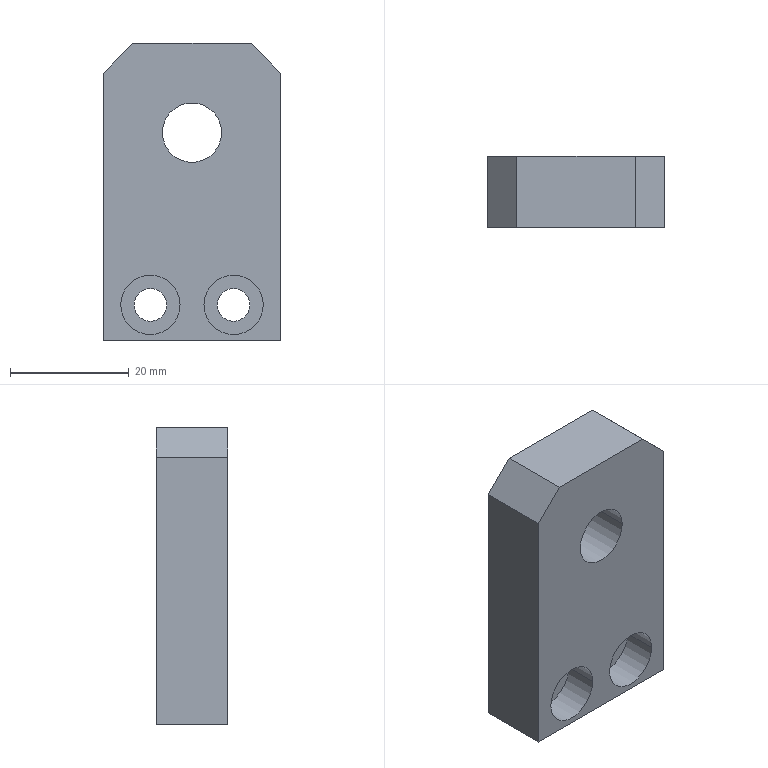Component | SolidWorks | XT-1-17-2-1 | 1 solid | 20 faces | box 29.9 x 12 x 50 mm | volume 15503 mm3 | cylinder 10 | plane 10 | commonest cylinder face diameters 10 x6 5.5 x4
build123d program:
from build123d import *

# Parameters (mm, degrees)
SKETCH1_W                                            = 29.9
SKETCH1_H                                            = 50
BOSS_EXTRUDE1_DEPTH                                  = 12
HOLE_SIZE_ACCORDING_TO_THE_TYPE_OF_HEXAG_D           = 5.5
HOLE_SIZE_ACCORDING_TO_THE_TYPE_OF_HEXAG_CBORE_D     = 10
HOLE_SIZE_ACCORDING_TO_THE_TYPE_OF_HEXAG_CBORE_DEPTH = 5.7
M10_TAPPED_HOLE1_D                                   = 10
CHAMFER1_SIZE                                        = 5


with BuildPart() as part:
    # Sketch1 → Boss-Extrude1 (new body)
    with BuildSketch(Plane.XY):
        Rectangle(SKETCH1_W, SKETCH1_H)
    extrude(amount=BOSS_EXTRUDE1_DEPTH)

    # Hole Size according to the type of Hexag (through all)
    with Locations(Plane.XY.offset(12)):
        with Locations((-7, 19), (7, 19)):
            CounterBoreHole(HOLE_SIZE_ACCORDING_TO_THE_TYPE_OF_HEXAG_D / 2, HOLE_SIZE_ACCORDING_TO_THE_TYPE_OF_HEXAG_CBORE_D / 2, HOLE_SIZE_ACCORDING_TO_THE_TYPE_OF_HEXAG_CBORE_DEPTH)

    # M10 Tapped Hole1 (through all)
    with Locations(Plane(origin=(0, 0, 0), x_dir=(-1, 0, 0), z_dir=(0, 0, -1))):
        with Locations((0, -10)):
            Hole(M10_TAPPED_HOLE1_D / 2)

    # Chamfer1
    chamfer1_edges = [part.edges().sort_by_distance(p)[0] for p in [
        (14.95, -25, 6),
        (-14.95, -25, 6),
    ]]
    chamfer(chamfer1_edges, length=CHAMFER1_SIZE)


solid = part.part

# Placed as in the assembly
solid = solid.moved(Location((647.283, -253.615, -141), (90, 0, -180)))
STEP:
#1=COLOUR_RGB('',0.7922,0.8196,0.9333);
#2=FILL_AREA_STYLE_COLOUR('',#1);
#3=FILL_AREA_STYLE('',(#2));
#4=SURFACE_STYLE_FILL_AREA(#3);
#5=SURFACE_SIDE_STYLE('',(#4));
#6=SURFACE_STYLE_USAGE(.BOTH.,#5);
#7=PRESENTATION_STYLE_ASSIGNMENT((#6));
#8=CARTESIAN_POINT('',(25.287,-10.457,-5.157));
#9=VERTEX_POINT('',#8);
#10=CARTESIAN_POINT('',(25.68,-10.457,-5.157));
#11=VERTEX_POINT('',#10);
#12=CARTESIAN_POINT('',(25.484,-10.457,-5.157));
#13=DIRECTION('',(0.,1.,0.));
#14=DIRECTION('',(1.,0.,0.));
#15=AXIS2_PLACEMENT_3D('',#12,#13,#14);
#16=CIRCLE('',#15,0.1969);
#17=EDGE_CURVE('',#9,#11,#16,.T.);
#18=ORIENTED_EDGE('',*,*,#17,.F.);
#19=CARTESIAN_POINT('',(25.287,-9.985,-5.157));
#20=VERTEX_POINT('',#19);
#21=CARTESIAN_POINT('',(25.287,-9.985,-5.157));
#22=DIRECTION('',(0.,1.,0.));
#23=VECTOR('',#22,39.37);
#24=LINE('',#21,#23);
#25=EDGE_CURVE('',#9,#20,#24,.T.);
#26=ORIENTED_EDGE('',*,*,#25,.T.);
#27=CARTESIAN_POINT('',(25.68,-9.985,-5.157));
#28=VERTEX_POINT('',#27);
#29=CARTESIAN_POINT('',(25.484,-9.985,-5.157));
#30=DIRECTION('',(0.,1.,0.));
#31=DIRECTION('',(1.,0.,0.));
#32=AXIS2_PLACEMENT_3D('',#29,#30,#31);
#33=CIRCLE('',#32,0.1969);
#34=EDGE_CURVE('',#20,#28,#33,.T.);
#35=ORIENTED_EDGE('',*,*,#34,.T.);
#36=CARTESIAN_POINT('',(25.68,-9.985,-5.157));
#37=DIRECTION('',(0.,1.,0.));
#38=VECTOR('',#37,39.37);
#39=LINE('',#36,#38);
#40=EDGE_CURVE('',#11,#28,#39,.T.);
#41=ORIENTED_EDGE('',*,*,#40,.F.);
#42=EDGE_LOOP('',(#18,#26,#35,#41));
#43=FACE_OUTER_BOUND('',#42,.T.);
#44=CARTESIAN_POINT('',(25.484,-9.985,-5.157));
#45=DIRECTION('',(0.,1.,0.));
#46=DIRECTION('',(1.,0.,0.));
#47=AXIS2_PLACEMENT_3D('',#44,#45,#46);
#48=CYLINDRICAL_SURFACE('',#47,0.1969);
#49=ADVANCED_FACE('',(#43),#48,.F.);
#50=CARTESIAN_POINT('',(25.956,-10.233,-6.299));
#51=VERTEX_POINT('',#50);
#52=CARTESIAN_POINT('',(25.562,-10.233,-6.299));
#53=VERTEX_POINT('',#52);
#54=CARTESIAN_POINT('',(25.759,-10.233,-6.299));
#55=DIRECTION('',(-0.,-1.,-0.));
#56=DIRECTION('',(-1.,0.,0.));
#57=AXIS2_PLACEMENT_3D('',#54,#55,#56);
#58=CIRCLE('',#57,0.1969);
#59=EDGE_CURVE('',#51,#53,#58,.T.);
#60=ORIENTED_EDGE('',*,*,#59,.F.);
#61=CARTESIAN_POINT('',(25.956,-10.457,-6.299));
#62=VERTEX_POINT('',#61);
#63=CARTESIAN_POINT('',(25.956,-10.457,-6.299));
#64=DIRECTION('',(-0.,-1.,-0.));
#65=VECTOR('',#64,39.37);
#66=LINE('',#63,#65);
#67=EDGE_CURVE('',#51,#62,#66,.T.);
#68=ORIENTED_EDGE('',*,*,#67,.T.);
#69=CARTESIAN_POINT('',(25.562,-10.457,-6.299));
#70=VERTEX_POINT('',#69);
#71=CARTESIAN_POINT('',(25.759,-10.457,-6.299));
#72=DIRECTION('',(-0.,-1.,-0.));
#73=DIRECTION('',(-1.,0.,0.));
#74=AXIS2_PLACEMENT_3D('',#71,#72,#73);
#75=CIRCLE('',#74,0.1969);
#76=EDGE_CURVE('',#62,#70,#75,.T.);
#77=ORIENTED_EDGE('',*,*,#76,.T.);
#78=CARTESIAN_POINT('',(25.562,-10.457,-6.299));
#79=DIRECTION('',(-0.,-1.,-0.));
#80=VECTOR('',#79,39.37);
#81=LINE('',#78,#80);
#82=EDGE_CURVE('',#53,#70,#81,.T.);
#83=ORIENTED_EDGE('',*,*,#82,.F.);
#84=EDGE_LOOP('',(#60,#68,#77,#83));
#85=FACE_OUTER_BOUND('',#84,.T.);
#86=CARTESIAN_POINT('',(25.759,-10.457,-6.299));
#87=DIRECTION('',(-0.,-1.,-0.));
#88=DIRECTION('',(-1.,0.,0.));
#89=AXIS2_PLACEMENT_3D('',#86,#87,#88);
#90=CYLINDRICAL_SURFACE('',#89,0.1969);
#91=ADVANCED_FACE('',(#85),#90,.F.);
#92=CARTESIAN_POINT('',(25.867,-9.985,-6.299));
#93=VERTEX_POINT('',#92);
#94=CARTESIAN_POINT('',(25.651,-9.985,-6.299));
#95=VERTEX_POINT('',#94);
#96=CARTESIAN_POINT('',(25.759,-9.985,-6.299));
#97=DIRECTION('',(-0.,-1.,-0.));
#98=DIRECTION('',(-1.,0.,0.));
#99=AXIS2_PLACEMENT_3D('',#96,#97,#98);
#100=CIRCLE('',#99,0.1083);
#101=EDGE_CURVE('',#93,#95,#100,.T.);
#102=ORIENTED_EDGE('',*,*,#101,.F.);
#103=CARTESIAN_POINT('',(25.867,-10.233,-6.299));
#104=VERTEX_POINT('',#103);
#105=CARTESIAN_POINT('',(25.867,-10.457,-6.299));
#106=DIRECTION('',(-0.,-1.,-0.));
#107=VECTOR('',#106,39.37);
#108=LINE('',#105,#107);
#109=EDGE_CURVE('',#93,#104,#108,.T.);
#110=ORIENTED_EDGE('',*,*,#109,.T.);
#111=CARTESIAN_POINT('',(25.651,-10.233,-6.299));
#112=VERTEX_POINT('',#111);
#113=CARTESIAN_POINT('',(25.759,-10.233,-6.299));
#114=DIRECTION('',(-0.,-1.,-0.));
#115=DIRECTION('',(-1.,0.,0.));
#116=AXIS2_PLACEMENT_3D('',#113,#114,#115);
#117=CIRCLE('',#116,0.1083);
#118=EDGE_CURVE('',#104,#112,#117,.T.);
#119=ORIENTED_EDGE('',*,*,#118,.T.);
#120=CARTESIAN_POINT('',(25.651,-10.457,-6.299));
#121=DIRECTION('',(-0.,-1.,-0.));
#122=VECTOR('',#121,39.37);
#123=LINE('',#120,#122);
#124=EDGE_CURVE('',#95,#112,#123,.T.);
#125=ORIENTED_EDGE('',*,*,#124,.F.);
#126=EDGE_LOOP('',(#102,#110,#119,#125));
#127=FACE_OUTER_BOUND('',#126,.T.);
#128=CARTESIAN_POINT('',(25.759,-10.457,-6.299));
#129=DIRECTION('',(-0.,-1.,-0.));
#130=DIRECTION('',(-1.,0.,0.));
#131=AXIS2_PLACEMENT_3D('',#128,#129,#130);
#132=CYLINDRICAL_SURFACE('',#131,0.1083);
#133=ADVANCED_FACE('',(#127),#132,.F.);
#134=CARTESIAN_POINT('',(25.405,-10.233,-6.299));
#135=VERTEX_POINT('',#134);
#136=CARTESIAN_POINT('',(25.011,-10.233,-6.299));
#137=VERTEX_POINT('',#136);
#138=CARTESIAN_POINT('',(25.208,-10.233,-6.299));
#139=DIRECTION('',(-0.,-1.,-0.));
#140=DIRECTION('',(-1.,0.,0.));
#141=AXIS2_PLACEMENT_3D('',#138,#139,#140);
#142=CIRCLE('',#141,0.1969);
#143=EDGE_CURVE('',#135,#137,#142,.T.);
#144=ORIENTED_EDGE('',*,*,#143,.F.);
#145=CARTESIAN_POINT('',(25.405,-10.457,-6.299));
#146=VERTEX_POINT('',#145);
#147=CARTESIAN_POINT('',(25.405,-10.457,-6.299));
#148=DIRECTION('',(-0.,-1.,-0.));
#149=VECTOR('',#148,39.37);
#150=LINE('',#147,#149);
#151=EDGE_CURVE('',#135,#146,#150,.T.);
#152=ORIENTED_EDGE('',*,*,#151,.T.);
#153=CARTESIAN_POINT('',(25.011,-10.457,-6.299));
#154=VERTEX_POINT('',#153);
#155=CARTESIAN_POINT('',(25.208,-10.457,-6.299));
#156=DIRECTION('',(-0.,-1.,-0.));
#157=DIRECTION('',(-1.,0.,0.));
#158=AXIS2_PLACEMENT_3D('',#155,#156,#157);
#159=CIRCLE('',#158,0.1969);
#160=EDGE_CURVE('',#146,#154,#159,.T.);
#161=ORIENTED_EDGE('',*,*,#160,.T.);
#162=CARTESIAN_POINT('',(25.011,-10.457,-6.299));
#163=DIRECTION('',(-0.,-1.,-0.));
#164=VECTOR('',#163,39.37);
#165=LINE('',#162,#164);
#166=EDGE_CURVE('',#137,#154,#165,.T.);
#167=ORIENTED_EDGE('',*,*,#166,.F.);
#168=EDGE_LOOP('',(#144,#152,#161,#167));
#169=FACE_OUTER_BOUND('',#168,.T.);
#170=CARTESIAN_POINT('',(25.208,-10.457,-6.299));
#171=DIRECTION('',(-0.,-1.,-0.));
#172=DIRECTION('',(-1.,0.,0.));
#173=AXIS2_PLACEMENT_3D('',#170,#171,#172);
#174=CYLINDRICAL_SURFACE('',#173,0.1969);
#175=ADVANCED_FACE('',(#169),#174,.F.);
#176=CARTESIAN_POINT('',(25.316,-9.985,-6.299));
#177=VERTEX_POINT('',#176);
#178=CARTESIAN_POINT('',(25.1,-9.985,-6.299));
#179=VERTEX_POINT('',#178);
#180=CARTESIAN_POINT('',(25.208,-9.985,-6.299));
#181=DIRECTION('',(-0.,-1.,-0.));
#182=DIRECTION('',(-1.,0.,0.));
#183=AXIS2_PLACEMENT_3D('',#180,#181,#182);
#184=CIRCLE('',#183,0.1083);
#185=EDGE_CURVE('',#177,#179,#184,.T.);
#186=ORIENTED_EDGE('',*,*,#185,.F.);
#187=CARTESIAN_POINT('',(25.316,-10.233,-6.299));
#188=VERTEX_POINT('',#187);
#189=CARTESIAN_POINT('',(25.316,-10.457,-6.299));
#190=DIRECTION('',(-0.,-1.,-0.));
#191=VECTOR('',#190,39.37);
#192=LINE('',#189,#191);
#193=EDGE_CURVE('',#177,#188,#192,.T.);
#194=ORIENTED_EDGE('',*,*,#193,.T.);
#195=CARTESIAN_POINT('',(25.1,-10.233,-6.299));
#196=VERTEX_POINT('',#195);
#197=CARTESIAN_POINT('',(25.208,-10.233,-6.299));
#198=DIRECTION('',(-0.,-1.,-0.));
#199=DIRECTION('',(-1.,0.,0.));
#200=AXIS2_PLACEMENT_3D('',#197,#198,#199);
#201=CIRCLE('',#200,0.1083);
#202=EDGE_CURVE('',#188,#196,#201,.T.);
#203=ORIENTED_EDGE('',*,*,#202,.T.);
#204=CARTESIAN_POINT('',(25.1,-10.457,-6.299));
#205=DIRECTION('',(-0.,-1.,-0.));
#206=VECTOR('',#205,39.37);
#207=LINE('',#204,#206);
#208=EDGE_CURVE('',#179,#196,#207,.T.);
#209=ORIENTED_EDGE('',*,*,#208,.F.);
#210=EDGE_LOOP('',(#186,#194,#203,#209));
#211=FACE_OUTER_BOUND('',#210,.T.);
#212=CARTESIAN_POINT('',(25.208,-10.457,-6.299));
#213=DIRECTION('',(-0.,-1.,-0.));
#214=DIRECTION('',(-1.,0.,0.));
#215=AXIS2_PLACEMENT_3D('',#212,#213,#214);
#216=CYLINDRICAL_SURFACE('',#215,0.1083);
#217=ADVANCED_FACE('',(#211),#216,.F.);
#218=CARTESIAN_POINT('',(24.895,-10.457,-4.764));
#219=VERTEX_POINT('',#218);
#220=CARTESIAN_POINT('',(24.895,-10.457,-6.535));
#221=VERTEX_POINT('',#220);
#222=CARTESIAN_POINT('',(24.895,-10.457,-4.567));
#223=DIRECTION('',(0.,-0.,-1.));
#224=VECTOR('',#223,39.37);
#225=LINE('',#222,#224);
#226=EDGE_CURVE('',#219,#221,#225,.T.);
#227=ORIENTED_EDGE('',*,*,#226,.F.);
#228=CARTESIAN_POINT('',(24.895,-9.985,-4.764));
#229=VERTEX_POINT('',#228);
#230=CARTESIAN_POINT('',(24.895,-10.457,-4.764));
#231=DIRECTION('',(0.,1.,0.));
#232=VECTOR('',#231,39.37);
#233=LINE('',#230,#232);
#234=EDGE_CURVE('',#219,#229,#233,.T.);
#235=ORIENTED_EDGE('',*,*,#234,.T.);
#236=CARTESIAN_POINT('',(24.895,-9.985,-6.535));
#237=VERTEX_POINT('',#236);
#238=CARTESIAN_POINT('',(24.895,-9.985,-4.567));
#239=DIRECTION('',(0.,-0.,-1.));
#240=VECTOR('',#239,39.37);
#241=LINE('',#238,#240);
#242=EDGE_CURVE('',#229,#237,#241,.T.);
#243=ORIENTED_EDGE('',*,*,#242,.T.);
#244=CARTESIAN_POINT('',(24.895,-10.457,-6.535));
#245=DIRECTION('',(0.,1.,0.));
#246=VECTOR('',#245,39.37);
#247=LINE('',#244,#246);
#248=EDGE_CURVE('',#221,#237,#247,.T.);
#249=ORIENTED_EDGE('',*,*,#248,.F.);
#250=EDGE_LOOP('',(#227,#235,#243,#249));
#251=FACE_OUTER_BOUND('',#250,.T.);
#252=CARTESIAN_POINT('',(24.895,-10.457,-4.567));
#253=DIRECTION('',(1.,-0.,0.));
#254=DIRECTION('',(-0.,-1.,-0.));
#255=AXIS2_PLACEMENT_3D('',#252,#253,#254);
#256=PLANE('',#255);
#257=ADVANCED_FACE('',(#251),#256,.F.);
#258=CARTESIAN_POINT('',(26.072,-9.985,-6.535));
#259=VERTEX_POINT('',#258);
#260=CARTESIAN_POINT('',(26.072,-9.985,-6.535));
#261=DIRECTION('',(1.,-0.,0.));
#262=VECTOR('',#261,39.37);
#263=LINE('',#260,#262);
#264=EDGE_CURVE('',#237,#259,#263,.T.);
#265=ORIENTED_EDGE('',*,*,#264,.T.);
#266=CARTESIAN_POINT('',(26.072,-10.457,-6.535));
#267=VERTEX_POINT('',#266);
#268=CARTESIAN_POINT('',(26.072,-10.457,-6.535));
#269=DIRECTION('',(0.,1.,0.));
#270=VECTOR('',#269,39.37);
#271=LINE('',#268,#270);
#272=EDGE_CURVE('',#267,#259,#271,.T.);
#273=ORIENTED_EDGE('',*,*,#272,.F.);
#274=CARTESIAN_POINT('',(26.072,-10.457,-6.535));
#275=DIRECTION('',(1.,-0.,0.));
#276=VECTOR('',#275,39.37);
#277=LINE('',#274,#276);
#278=EDGE_CURVE('',#221,#267,#277,.T.);
#279=ORIENTED_EDGE('',*,*,#278,.F.);
#280=ORIENTED_EDGE('',*,*,#248,.T.);
#281=EDGE_LOOP('',(#265,#273,#279,#280));
#282=FACE_OUTER_BOUND('',#281,.T.);
#283=CARTESIAN_POINT('',(26.072,-10.457,-6.535));
#284=DIRECTION('',(-0.,0.,1.));
#285=DIRECTION('',(0.,1.,0.));
#286=AXIS2_PLACEMENT_3D('',#283,#284,#285);
#287=PLANE('',#286);
#288=ADVANCED_FACE('',(#282),#287,.F.);
#289=CARTESIAN_POINT('',(26.072,-9.985,-4.764));
#290=VERTEX_POINT('',#289);
#291=CARTESIAN_POINT('',(26.072,-9.985,-4.567));
#292=DIRECTION('',(-0.,0.,1.));
#293=VECTOR('',#292,39.37);
#294=LINE('',#291,#293);
#295=EDGE_CURVE('',#259,#290,#294,.T.);
#296=ORIENTED_EDGE('',*,*,#295,.T.);
#297=CARTESIAN_POINT('',(26.072,-10.457,-4.764));
#298=VERTEX_POINT('',#297);
#299=CARTESIAN_POINT('',(26.072,-10.457,-4.764));
#300=DIRECTION('',(-0.,-1.,-0.));
#301=VECTOR('',#300,39.37);
#302=LINE('',#299,#301);
#303=EDGE_CURVE('',#290,#298,#302,.T.);
#304=ORIENTED_EDGE('',*,*,#303,.T.);
#305=CARTESIAN_POINT('',(26.072,-10.457,-4.567));
#306=DIRECTION('',(-0.,0.,1.));
#307=VECTOR('',#306,39.37);
#308=LINE('',#305,#307);
#309=EDGE_CURVE('',#267,#298,#308,.T.);
#310=ORIENTED_EDGE('',*,*,#309,.F.);
#311=ORIENTED_EDGE('',*,*,#272,.T.);
#312=EDGE_LOOP('',(#296,#304,#310,#311));
#313=FACE_OUTER_BOUND('',#312,.T.);
#314=CARTESIAN_POINT('',(26.072,-10.457,-4.567));
#315=DIRECTION('',(-1.,0.,-0.));
#316=DIRECTION('',(0.,1.,0.));
#317=AXIS2_PLACEMENT_3D('',#314,#315,#316);
#318=PLANE('',#317);
#319=ADVANCED_FACE('',(#313),#318,.F.);
#320=CARTESIAN_POINT('',(25.875,-9.985,-4.567));
#321=VERTEX_POINT('',#320);
#322=CARTESIAN_POINT('',(25.092,-9.985,-4.567));
#323=VERTEX_POINT('',#322);
#324=CARTESIAN_POINT('',(26.072,-9.985,-4.567));
#325=DIRECTION('',(-1.,0.,-0.));
#326=VECTOR('',#325,39.37);
#327=LINE('',#324,#326);
#328=EDGE_CURVE('',#321,#323,#327,.T.);
#329=ORIENTED_EDGE('',*,*,#328,.T.);
#330=CARTESIAN_POINT('',(25.092,-10.457,-4.567));
#331=VERTEX_POINT('',#330);
#332=CARTESIAN_POINT('',(25.092,-10.457,-4.567));
#333=DIRECTION('',(-0.,-1.,-0.));
#334=VECTOR('',#333,39.37);
#335=LINE('',#332,#334);
#336=EDGE_CURVE('',#323,#331,#335,.T.);
#337=ORIENTED_EDGE('',*,*,#336,.T.);
#338=CARTESIAN_POINT('',(25.875,-10.457,-4.567));
#339=VERTEX_POINT('',#338);
#340=CARTESIAN_POINT('',(26.072,-10.457,-4.567));
#341=DIRECTION('',(-1.,0.,-0.));
#342=VECTOR('',#341,39.37);
#343=LINE('',#340,#342);
#344=EDGE_CURVE('',#339,#331,#343,.T.);
#345=ORIENTED_EDGE('',*,*,#344,.F.);
#346=CARTESIAN_POINT('',(25.875,-10.457,-4.567));
#347=DIRECTION('',(0.,1.,0.));
#348=VECTOR('',#347,39.37);
#349=LINE('',#346,#348);
#350=EDGE_CURVE('',#339,#321,#349,.T.);
#351=ORIENTED_EDGE('',*,*,#350,.T.);
#352=EDGE_LOOP('',(#329,#337,#345,#351));
#353=FACE_OUTER_BOUND('',#352,.T.);
#354=CARTESIAN_POINT('',(26.072,-10.457,-4.567));
#355=DIRECTION('',(0.,-0.,-1.));
#356=DIRECTION('',(-0.,-1.,-0.));
#357=AXIS2_PLACEMENT_3D('',#354,#355,#356);
#358=PLANE('',#357);
#359=ADVANCED_FACE('',(#353),#358,.F.);
#360=CARTESIAN_POINT('',(25.484,-10.457,-5.157));
#361=DIRECTION('',(0.,1.,0.));
#362=DIRECTION('',(1.,0.,0.));
#363=AXIS2_PLACEMENT_3D('',#360,#361,#362);
#364=CIRCLE('',#363,0.1969);
#365=EDGE_CURVE('',#11,#9,#364,.T.);
#366=ORIENTED_EDGE('',*,*,#365,.T.);
#367=ORIENTED_EDGE('',*,*,#17,.T.);
#368=EDGE_LOOP('',(#366,#367));
#369=FACE_BOUND('',#368,.T.);
#370=CARTESIAN_POINT('',(25.759,-10.457,-6.299));
#371=DIRECTION('',(-0.,-1.,-0.));
#372=DIRECTION('',(-1.,0.,0.));
#373=AXIS2_PLACEMENT_3D('',#370,#371,#372);
#374=CIRCLE('',#373,0.1969);
#375=EDGE_CURVE('',#70,#62,#374,.T.);
#376=ORIENTED_EDGE('',*,*,#375,.F.);
#377=ORIENTED_EDGE('',*,*,#76,.F.);
#378=EDGE_LOOP('',(#376,#377));
#379=FACE_BOUND('',#378,.T.);
#380=CARTESIAN_POINT('',(25.208,-10.457,-6.299));
#381=DIRECTION('',(-0.,-1.,-0.));
#382=DIRECTION('',(-1.,0.,0.));
#383=AXIS2_PLACEMENT_3D('',#380,#381,#382);
#384=CIRCLE('',#383,0.1969);
#385=EDGE_CURVE('',#154,#146,#384,.T.);
#386=ORIENTED_EDGE('',*,*,#385,.F.);
#387=ORIENTED_EDGE('',*,*,#160,.F.);
#388=EDGE_LOOP('',(#386,#387));
#389=FACE_BOUND('',#388,.T.);
#390=ORIENTED_EDGE('',*,*,#344,.T.);
#391=CARTESIAN_POINT('',(24.895,-10.457,-4.764));
#392=DIRECTION('',(-0.7071,0.,-0.7071));
#393=VECTOR('',#392,39.37);
#394=LINE('',#391,#393);
#395=EDGE_CURVE('',#331,#219,#394,.T.);
#396=ORIENTED_EDGE('',*,*,#395,.T.);
#397=ORIENTED_EDGE('',*,*,#226,.T.);
#398=ORIENTED_EDGE('',*,*,#278,.T.);
#399=ORIENTED_EDGE('',*,*,#309,.T.);
#400=CARTESIAN_POINT('',(25.875,-10.457,-4.567));
#401=DIRECTION('',(-0.7071,0.,0.7071));
#402=VECTOR('',#401,39.37);
#403=LINE('',#400,#402);
#404=EDGE_CURVE('',#298,#339,#403,.T.);
#405=ORIENTED_EDGE('',*,*,#404,.T.);
#406=EDGE_LOOP('',(#390,#396,#397,#398,#399,#405));
#407=FACE_OUTER_BOUND('',#406,.T.);
#408=CARTESIAN_POINT('',(24.895,-10.457,-6.535));
#409=DIRECTION('',(0.,1.,0.));
#410=DIRECTION('',(1.,-0.,0.));
#411=AXIS2_PLACEMENT_3D('',#408,#409,#410);
#412=PLANE('',#411);
#413=ADVANCED_FACE('',(#369,#379,#389,#407),#412,.F.);
#414=CARTESIAN_POINT('',(25.484,-9.985,-5.157));
#415=DIRECTION('',(0.,1.,0.));
#416=DIRECTION('',(1.,0.,0.));
#417=AXIS2_PLACEMENT_3D('',#414,#415,#416);
#418=CIRCLE('',#417,0.1969);
#419=EDGE_CURVE('',#28,#20,#418,.T.);
#420=ORIENTED_EDGE('',*,*,#419,.F.);
#421=ORIENTED_EDGE('',*,*,#34,.F.);
#422=EDGE_LOOP('',(#420,#421));
#423=FACE_BOUND('',#422,.T.);
#424=CARTESIAN_POINT('',(25.759,-9.985,-6.299));
#425=DIRECTION('',(-0.,-1.,-0.));
#426=DIRECTION('',(-1.,0.,0.));
#427=AXIS2_PLACEMENT_3D('',#424,#425,#426);
#428=CIRCLE('',#427,0.1083);
#429=EDGE_CURVE('',#95,#93,#428,.T.);
#430=ORIENTED_EDGE('',*,*,#429,.T.);
#431=ORIENTED_EDGE('',*,*,#101,.T.);
#432=EDGE_LOOP('',(#430,#431));
#433=FACE_BOUND('',#432,.T.);
#434=CARTESIAN_POINT('',(25.208,-9.985,-6.299));
#435=DIRECTION('',(-0.,-1.,-0.));
#436=DIRECTION('',(-1.,0.,0.));
#437=AXIS2_PLACEMENT_3D('',#434,#435,#436);
#438=CIRCLE('',#437,0.1083);
#439=EDGE_CURVE('',#179,#177,#438,.T.);
#440=ORIENTED_EDGE('',*,*,#439,.T.);
#441=ORIENTED_EDGE('',*,*,#185,.T.);
#442=EDGE_LOOP('',(#440,#441));
#443=FACE_BOUND('',#442,.T.);
#444=ORIENTED_EDGE('',*,*,#242,.F.);
#445=CARTESIAN_POINT('',(24.009,-9.985,-5.65));
#446=DIRECTION('',(0.7071,-0.,0.7071));
#447=VECTOR('',#446,39.37);
#448=LINE('',#445,#447);
#449=EDGE_CURVE('',#229,#323,#448,.T.);
#450=ORIENTED_EDGE('',*,*,#449,.T.);
#451=ORIENTED_EDGE('',*,*,#328,.F.);
#452=CARTESIAN_POINT('',(26.369,-9.985,-5.061));
#453=DIRECTION('',(0.7071,-0.,-0.7071));
#454=VECTOR('',#453,39.37);
#455=LINE('',#452,#454);
#456=EDGE_CURVE('',#321,#290,#455,.T.);
#457=ORIENTED_EDGE('',*,*,#456,.T.);
#458=ORIENTED_EDGE('',*,*,#295,.F.);
#459=ORIENTED_EDGE('',*,*,#264,.F.);
#460=EDGE_LOOP('',(#444,#450,#451,#457,#458,#459));
#461=FACE_OUTER_BOUND('',#460,.T.);
#462=CARTESIAN_POINT('',(24.895,-9.985,-6.535));
#463=DIRECTION('',(0.,1.,0.));
#464=DIRECTION('',(1.,-0.,0.));
#465=AXIS2_PLACEMENT_3D('',#462,#463,#464);
#466=PLANE('',#465);
#467=ADVANCED_FACE('',(#423,#433,#443,#461),#466,.T.);
#468=ORIENTED_EDGE('',*,*,#193,.F.);
#469=ORIENTED_EDGE('',*,*,#439,.F.);
#470=ORIENTED_EDGE('',*,*,#208,.T.);
#471=CARTESIAN_POINT('',(25.208,-10.233,-6.299));
#472=DIRECTION('',(-0.,-1.,-0.));
#473=DIRECTION('',(-1.,0.,0.));
#474=AXIS2_PLACEMENT_3D('',#471,#472,#473);
#475=CIRCLE('',#474,0.1083);
#476=EDGE_CURVE('',#196,#188,#475,.T.);
#477=ORIENTED_EDGE('',*,*,#476,.T.);
#478=EDGE_LOOP('',(#468,#469,#470,#477));
#479=FACE_OUTER_BOUND('',#478,.T.);
#480=CARTESIAN_POINT('',(25.208,-10.457,-6.299));
#481=DIRECTION('',(-0.,-1.,-0.));
#482=DIRECTION('',(-1.,0.,0.));
#483=AXIS2_PLACEMENT_3D('',#480,#481,#482);
#484=CYLINDRICAL_SURFACE('',#483,0.1083);
#485=ADVANCED_FACE('',(#479),#484,.F.);
#486=ORIENTED_EDGE('',*,*,#476,.F.);
#487=ORIENTED_EDGE('',*,*,#202,.F.);
#488=EDGE_LOOP('',(#486,#487));
#489=FACE_BOUND('',#488,.T.);
#490=CARTESIAN_POINT('',(25.208,-10.233,-6.299));
#491=DIRECTION('',(-0.,-1.,-0.));
#492=DIRECTION('',(-1.,0.,0.));
#493=AXIS2_PLACEMENT_3D('',#490,#491,#492);
#494=CIRCLE('',#493,0.1969);
#495=EDGE_CURVE('',#137,#135,#494,.T.);
#496=ORIENTED_EDGE('',*,*,#495,.T.);
#497=ORIENTED_EDGE('',*,*,#143,.T.);
#498=EDGE_LOOP('',(#496,#497));
#499=FACE_OUTER_BOUND('',#498,.T.);
#500=CARTESIAN_POINT('',(25.1,-10.233,-6.299));
#501=DIRECTION('',(0.,1.,0.));
#502=DIRECTION('',(1.,-0.,0.));
#503=AXIS2_PLACEMENT_3D('',#500,#501,#502);
#504=PLANE('',#503);
#505=ADVANCED_FACE('',(#489,#499),#504,.F.);
#506=ORIENTED_EDGE('',*,*,#151,.F.);
#507=ORIENTED_EDGE('',*,*,#495,.F.);
#508=ORIENTED_EDGE('',*,*,#166,.T.);
#509=ORIENTED_EDGE('',*,*,#385,.T.);
#510=EDGE_LOOP('',(#506,#507,#508,#509));
#511=FACE_OUTER_BOUND('',#510,.T.);
#512=CARTESIAN_POINT('',(25.208,-10.457,-6.299));
#513=DIRECTION('',(-0.,-1.,-0.));
#514=DIRECTION('',(-1.,0.,0.));
#515=AXIS2_PLACEMENT_3D('',#512,#513,#514);
#516=CYLINDRICAL_SURFACE('',#515,0.1969);
#517=ADVANCED_FACE('',(#511),#516,.F.);
#518=ORIENTED_EDGE('',*,*,#109,.F.);
#519=ORIENTED_EDGE('',*,*,#429,.F.);
#520=ORIENTED_EDGE('',*,*,#124,.T.);
#521=CARTESIAN_POINT('',(25.759,-10.233,-6.299));
#522=DIRECTION('',(-0.,-1.,-0.));
#523=DIRECTION('',(-1.,0.,0.));
#524=AXIS2_PLACEMENT_3D('',#521,#522,#523);
#525=CIRCLE('',#524,0.1083);
#526=EDGE_CURVE('',#112,#104,#525,.T.);
#527=ORIENTED_EDGE('',*,*,#526,.T.);
#528=EDGE_LOOP('',(#518,#519,#520,#527));
#529=FACE_OUTER_BOUND('',#528,.T.);
#530=CARTESIAN_POINT('',(25.759,-10.457,-6.299));
#531=DIRECTION('',(-0.,-1.,-0.));
#532=DIRECTION('',(-1.,0.,0.));
#533=AXIS2_PLACEMENT_3D('',#530,#531,#532);
#534=CYLINDRICAL_SURFACE('',#533,0.1083);
#535=ADVANCED_FACE('',(#529),#534,.F.);
#536=ORIENTED_EDGE('',*,*,#526,.F.);
#537=ORIENTED_EDGE('',*,*,#118,.F.);
#538=EDGE_LOOP('',(#536,#537));
#539=FACE_BOUND('',#538,.T.);
#540=CARTESIAN_POINT('',(25.759,-10.233,-6.299));
#541=DIRECTION('',(-0.,-1.,-0.));
#542=DIRECTION('',(-1.,0.,0.));
#543=AXIS2_PLACEMENT_3D('',#540,#541,#542);
#544=CIRCLE('',#543,0.1969);
#545=EDGE_CURVE('',#53,#51,#544,.T.);
#546=ORIENTED_EDGE('',*,*,#545,.T.);
#547=ORIENTED_EDGE('',*,*,#59,.T.);
#548=EDGE_LOOP('',(#546,#547));
#549=FACE_OUTER_BOUND('',#548,.T.);
#550=CARTESIAN_POINT('',(25.651,-10.233,-6.299));
#551=DIRECTION('',(0.,1.,0.));
#552=DIRECTION('',(1.,-0.,0.));
#553=AXIS2_PLACEMENT_3D('',#550,#551,#552);
#554=PLANE('',#553);
#555=ADVANCED_FACE('',(#539,#549),#554,.F.);
#556=ORIENTED_EDGE('',*,*,#67,.F.);
#557=ORIENTED_EDGE('',*,*,#545,.F.);
#558=ORIENTED_EDGE('',*,*,#82,.T.);
#559=ORIENTED_EDGE('',*,*,#375,.T.);
#560=EDGE_LOOP('',(#556,#557,#558,#559));
#561=FACE_OUTER_BOUND('',#560,.T.);
#562=CARTESIAN_POINT('',(25.759,-10.457,-6.299));
#563=DIRECTION('',(-0.,-1.,-0.));
#564=DIRECTION('',(-1.,0.,0.));
#565=AXIS2_PLACEMENT_3D('',#562,#563,#564);
#566=CYLINDRICAL_SURFACE('',#565,0.1969);
#567=ADVANCED_FACE('',(#561),#566,.F.);
#568=ORIENTED_EDGE('',*,*,#25,.F.);
#569=ORIENTED_EDGE('',*,*,#365,.F.);
#570=ORIENTED_EDGE('',*,*,#40,.T.);
#571=ORIENTED_EDGE('',*,*,#419,.T.);
#572=EDGE_LOOP('',(#568,#569,#570,#571));
#573=FACE_OUTER_BOUND('',#572,.T.);
#574=CARTESIAN_POINT('',(25.484,-9.985,-5.157));
#575=DIRECTION('',(0.,1.,0.));
#576=DIRECTION('',(1.,0.,0.));
#577=AXIS2_PLACEMENT_3D('',#574,#575,#576);
#578=CYLINDRICAL_SURFACE('',#577,0.1969);
#579=ADVANCED_FACE('',(#573),#578,.F.);
#580=ORIENTED_EDGE('',*,*,#395,.F.);
#581=ORIENTED_EDGE('',*,*,#336,.F.);
#582=ORIENTED_EDGE('',*,*,#449,.F.);
#583=ORIENTED_EDGE('',*,*,#234,.F.);
#584=EDGE_LOOP('',(#580,#581,#582,#583));
#585=FACE_OUTER_BOUND('',#584,.T.);
#586=CARTESIAN_POINT('',(24.895,-10.457,-4.764));
#587=DIRECTION('',(0.7071,-0.,-0.7071));
#588=DIRECTION('',(0.7071,-0.,0.7071));
#589=AXIS2_PLACEMENT_3D('',#586,#587,#588);
#590=PLANE('',#589);
#591=ADVANCED_FACE('',(#585),#590,.F.);
#592=ORIENTED_EDGE('',*,*,#404,.F.);
#593=ORIENTED_EDGE('',*,*,#303,.F.);
#594=ORIENTED_EDGE('',*,*,#456,.F.);
#595=ORIENTED_EDGE('',*,*,#350,.F.);
#596=EDGE_LOOP('',(#592,#593,#594,#595));
#597=FACE_OUTER_BOUND('',#596,.T.);
#598=CARTESIAN_POINT('',(25.875,-10.457,-4.567));
#599=DIRECTION('',(-0.7071,0.,-0.7071));
#600=DIRECTION('',(0.7071,-0.,-0.7071));
#601=AXIS2_PLACEMENT_3D('',#598,#599,#600);
#602=PLANE('',#601);
#603=ADVANCED_FACE('',(#597),#602,.F.);
#604=CLOSED_SHELL('',(#49,#91,#133,#175,#217,#257,#288,#319,#359,#413,#467,#485,#505,#517,#535,#555,#567,#579,#591,#603));
#605=MANIFOLD_SOLID_BREP('',#604);
#606=STYLED_ITEM('',(#7),#605);
#607=PRESENTATION_LAYER_ASSIGNMENT('','',(#606));
#608=CARTESIAN_POINT('',(0.,0.,0.));
#609=DIRECTION('',(0.,0.,1.));
#610=DIRECTION('',(1.,0.,0.));
#611=AXIS2_PLACEMENT_3D('',#608,#609,#610);
#612=(LENGTH_UNIT()NAMED_UNIT(*)SI_UNIT($,.METRE.));
#613=LENGTH_MEASURE_WITH_UNIT(LENGTH_MEASURE(0.0254),#612);
#614=DIMENSIONAL_EXPONENTS(1.,0.,0.,0.,0.,0.,0.);
#615=(CONVERSION_BASED_UNIT('',#613)LENGTH_UNIT()NAMED_UNIT(#614));
#616=UNCERTAINTY_MEASURE_WITH_UNIT(LENGTH_MEASURE(0.00001),#615,'','');
#617=(NAMED_UNIT(*)PLANE_ANGLE_UNIT()SI_UNIT($,.RADIAN.));
#618=(NAMED_UNIT(*)SI_UNIT($,.STERADIAN.)SOLID_ANGLE_UNIT());
#619=(GEOMETRIC_REPRESENTATION_CONTEXT(3)GLOBAL_UNCERTAINTY_ASSIGNED_CONTEXT((#616))GLOBAL_UNIT_ASSIGNED_CONTEXT((#615,#617,#618))REPRESENTATION_CONTEXT('',''));
#620=ADVANCED_BREP_SHAPE_REPRESENTATION('',(#605,#611),#619);
#621=(LENGTH_UNIT()NAMED_UNIT(*)SI_UNIT($,.METRE.));
#622=LENGTH_MEASURE_WITH_UNIT(LENGTH_MEASURE(0.0254),#621);
#623=DIMENSIONAL_EXPONENTS(1.,0.,0.,0.,0.,0.,0.);
#624=(CONVERSION_BASED_UNIT('',#622)LENGTH_UNIT()NAMED_UNIT(#623));
#625=UNCERTAINTY_MEASURE_WITH_UNIT(LENGTH_MEASURE(0.00001),#624,'','');
#626=(NAMED_UNIT(*)PLANE_ANGLE_UNIT()SI_UNIT($,.RADIAN.));
#627=(NAMED_UNIT(*)SI_UNIT($,.STERADIAN.)SOLID_ANGLE_UNIT());
#628=(GEOMETRIC_REPRESENTATION_CONTEXT(3)GLOBAL_UNCERTAINTY_ASSIGNED_CONTEXT((#625))GLOBAL_UNIT_ASSIGNED_CONTEXT((#624,#626,#627))REPRESENTATION_CONTEXT('',''));
#629=MECHANICAL_DESIGN_GEOMETRIC_PRESENTATION_REPRESENTATION('',(#606),#628);